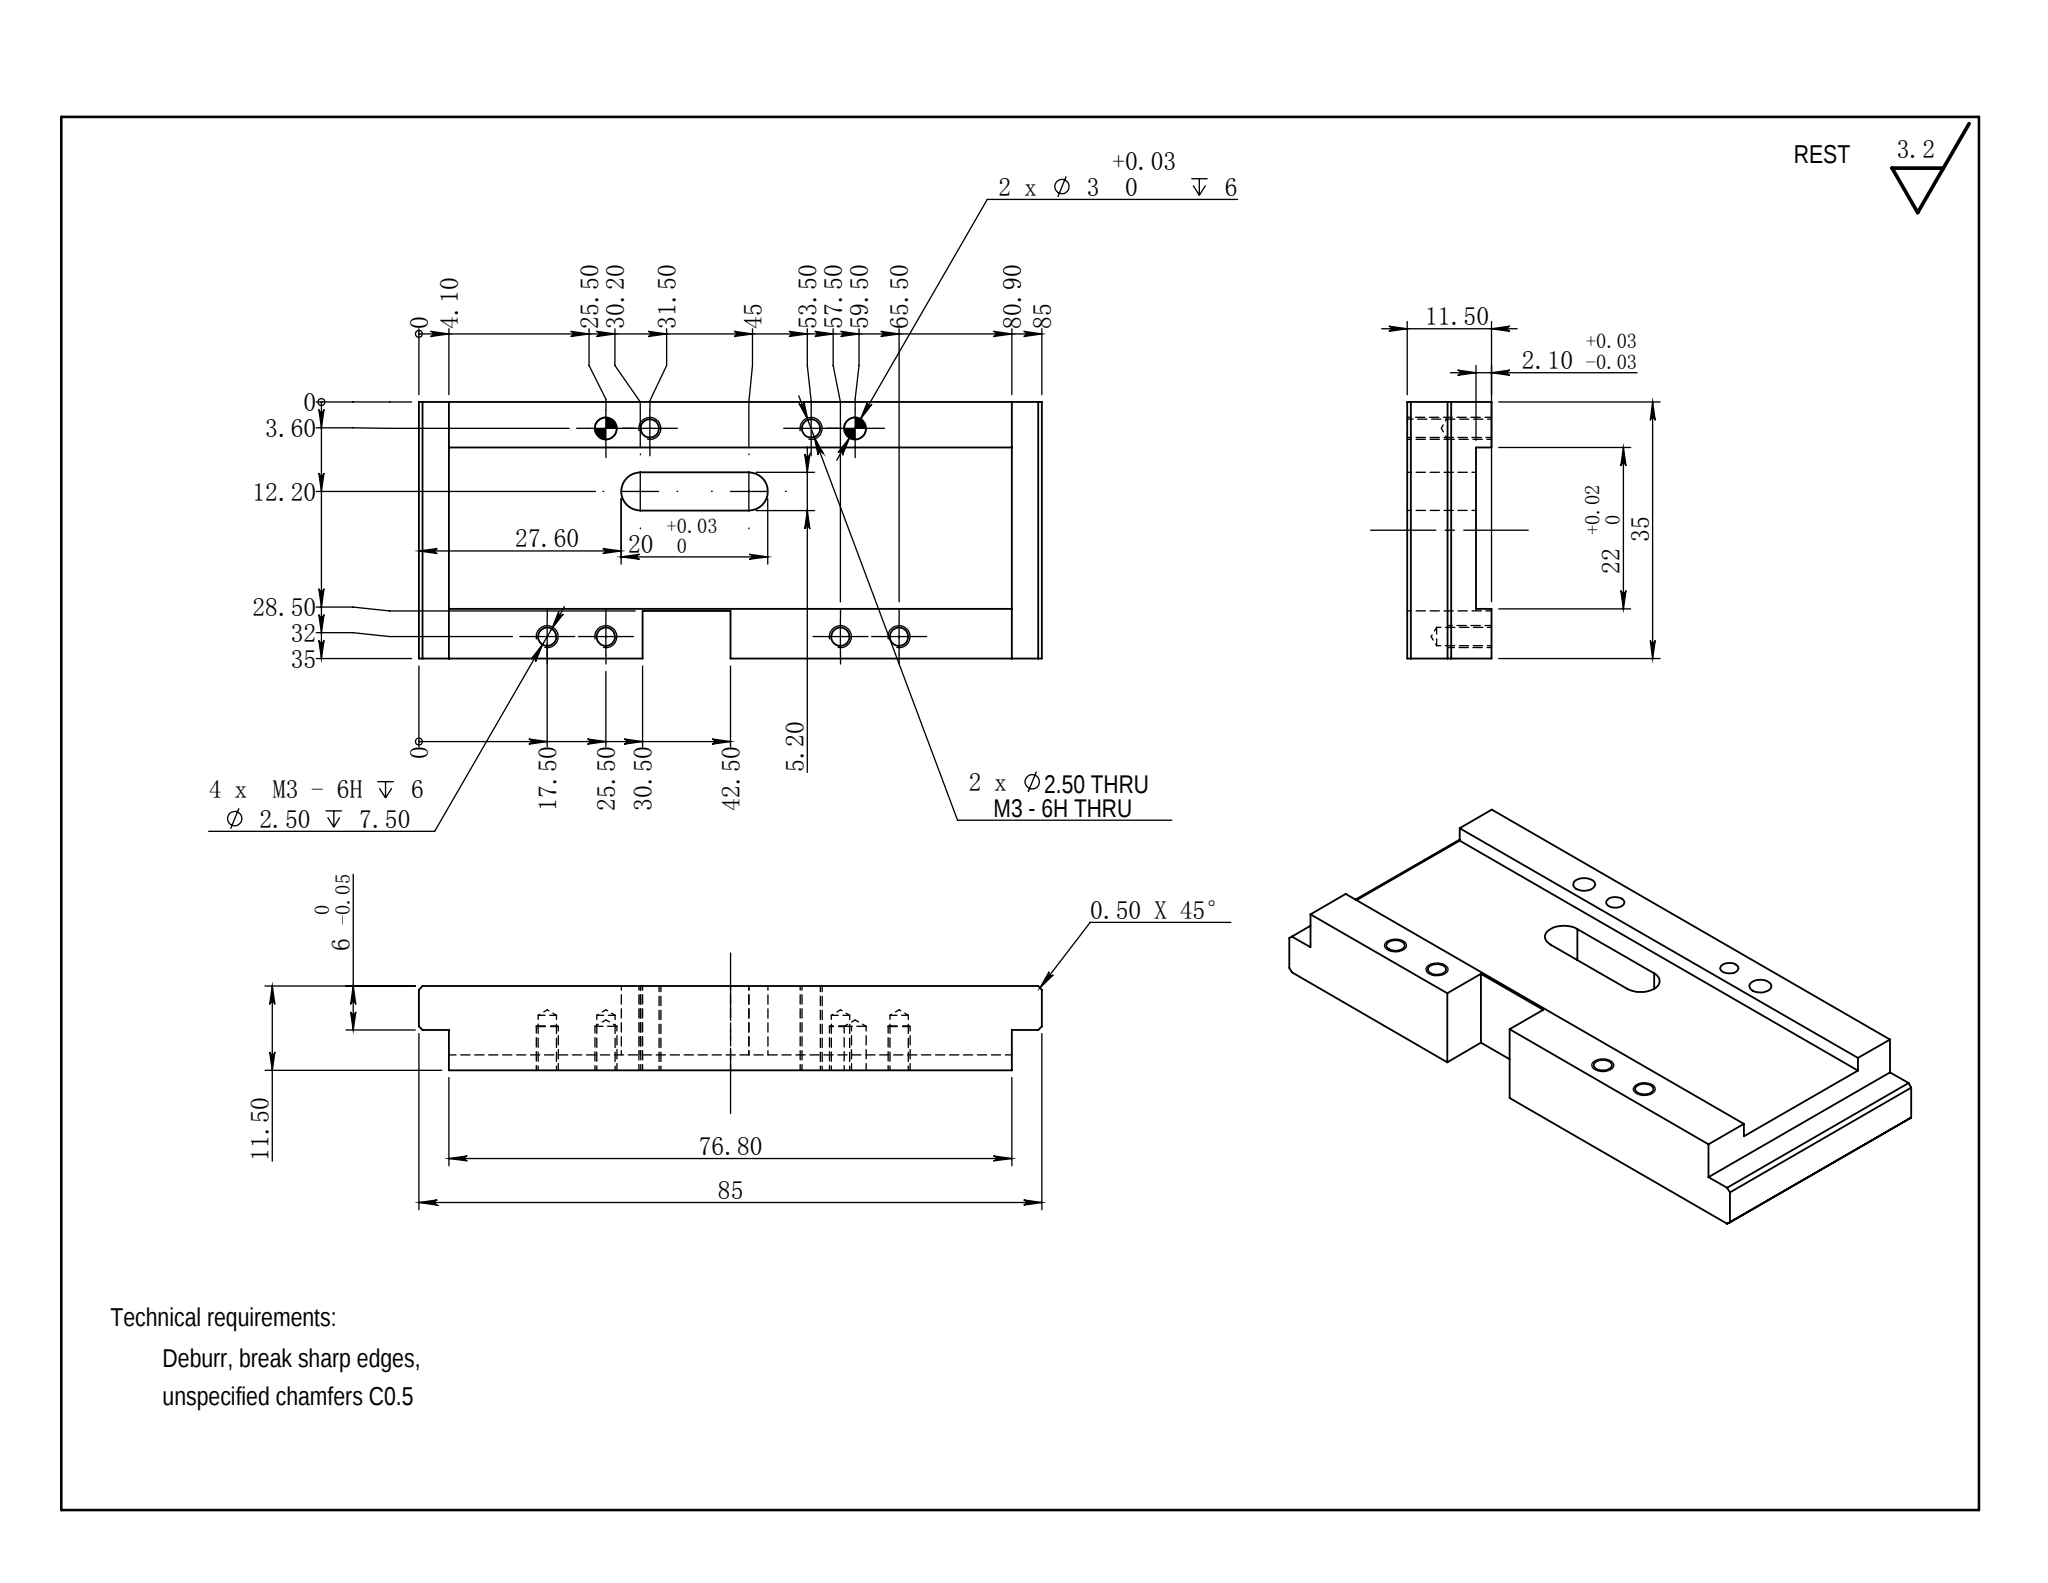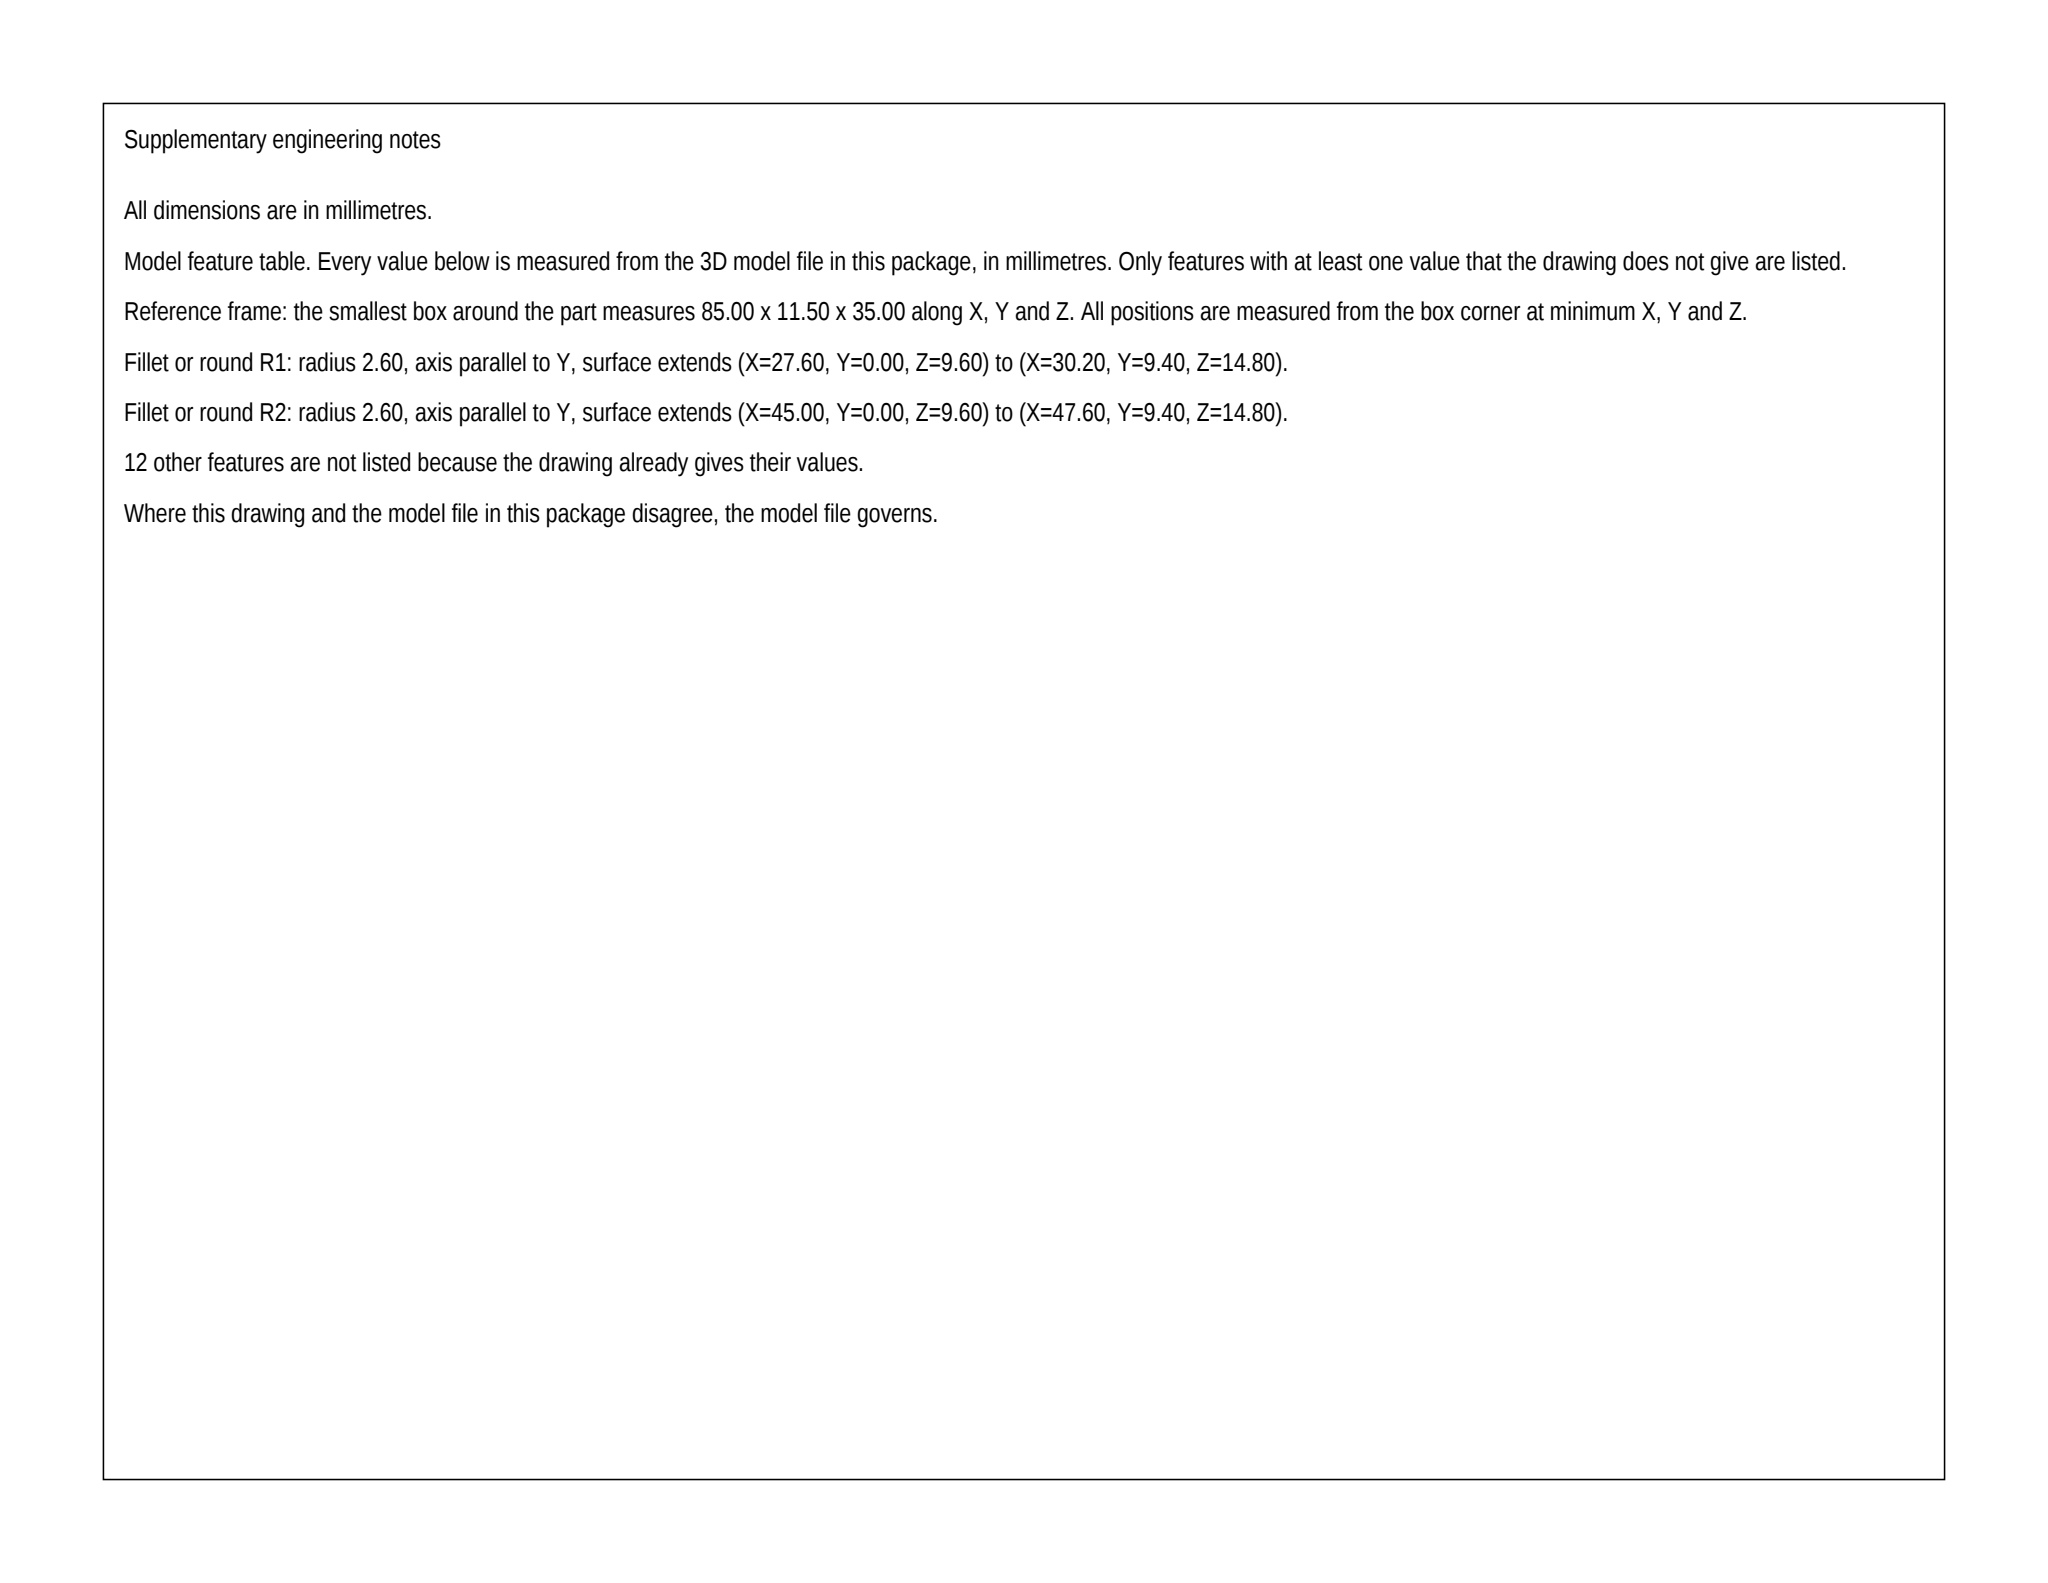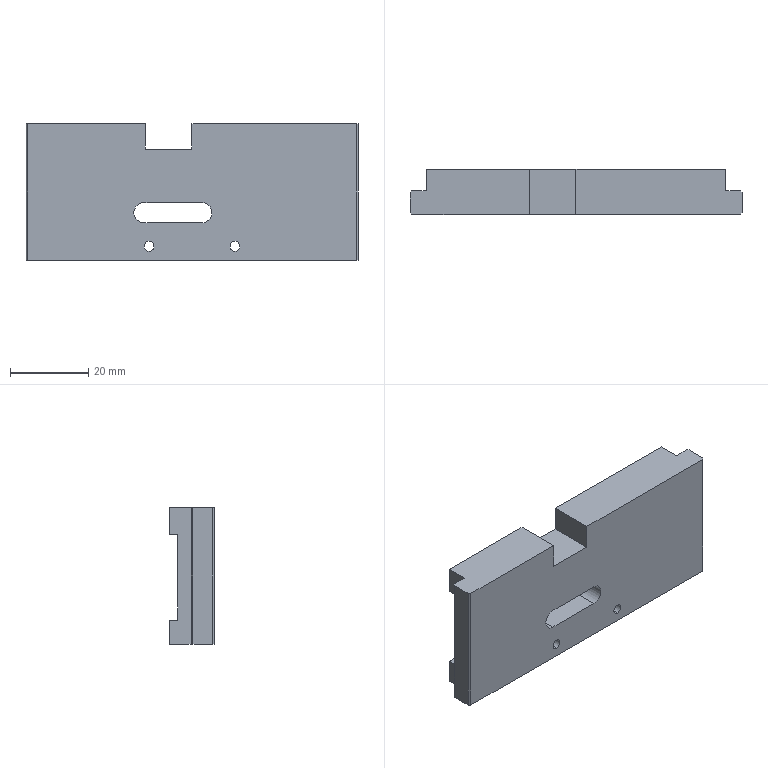Part | SolidWorks | mm | 1 solid | 54 faces | box 85 x 11.5 x 35 mm | volume 26894 mm3 | plane 24 | cylinder 18 | cone 12 | commonest cylinder face diameters 2.5 x12 3 x4 5.2 x2
Drawing notes:
22 GROOVE 6.20 FROM 0 DATUM EDGE, 6.80 FROM 35 EDGE | from the solid: z-planes 6.2 and 28.2 bound 22 wide groove in 35 width; 35-28.2=6.8
CENTRAL SLOT 5.20 WIDE, R2.60 ENDS, DP 9.40 | from the solid: 2x cyl Ø5.2 axis y at x=30.2 & 45.0, z=12.2, len 9.4; centers 14.8 apart = 20 OA
build123d program:
from build123d import *

# Parameters (mm, degrees)
SKETCH1_W                    = 85
SKETCH1_H                    = 35
BOSS_EXTRUDE1_DEPTH          = 11.5
SKETCH2_W                    = 85
SKETCH2_H                    = 22
CUT_EXTRUDE1_DEPTH           = 2.1
SKETCH4_W                    = 12
SKETCH4_H                    = 6.5
CUT_EXTRUDE3_DEPTH           = 48.379
M3_TAPPED_HOLE1_D            = 2.5
M3_TAPPED_HOLE1_DEPTH        = 7.5
M3_TAPPED_HOLE1_TIP          = 0.7511
M3_TAPPED_HOLE2_D            = 2.5
SKETCH27_W                   = 4.1
SKETCH27_H                   = 35
CUT_EXTRUDE9_DEPTH           = 5.5
F_3_0_3_DIAMETER_HOLE1_D     = 3
F_3_0_3_DIAMETER_HOLE1_DEPTH = 6
F_3_0_3_DIAMETER_HOLE1_TIP   = 0.866
SKETCH30_R                   = 2.6
CUT_EXTRUDE10_DEPTH          = 47.913
CHAMFER3_SIZE                = 0.5
CUT_EXTRUDE12_REACH          = 48.913


with BuildPart() as part:
    # Sketch1 → Boss-Extrude1 (new body)
    with BuildSketch(Plane(origin=(0, 0, 0), x_dir=(1, 0, 0), z_dir=(0, 1, 0))):
        Rectangle(SKETCH1_W, SKETCH1_H)
    extrude(amount=BOSS_EXTRUDE1_DEPTH)

    # Sketch2 → Cut-Extrude1 (cut)
    with BuildSketch(Plane(origin=(0, 11.5, 0), x_dir=(1, 0, 0), z_dir=(0, 1, 0))):
        with Locations((0, 0.3)):
            Rectangle(SKETCH2_W, SKETCH2_H)
    extrude(amount=-CUT_EXTRUDE1_DEPTH, mode=Mode.SUBTRACT)

    # Sketch4 → Cut-Extrude3 (cut, through all)
    with BuildSketch(Plane(origin=(0, 11.5, 0), x_dir=(1, 0, 0), z_dir=(0, 1, 0))):
        with Locations((-6, -14.25)):
            Rectangle(SKETCH4_W, SKETCH4_H)
    extrude(amount=-CUT_EXTRUDE3_DEPTH, mode=Mode.SUBTRACT)

    # M3 Tapped Hole1
    with Locations(Plane(origin=(0, 11.5, 0), x_dir=(1, 0, 0), z_dir=(0, 1, 0))):
        with Locations((-25, -14.5), (-17, -14.5), (15, -14.5), (23, -14.5)):
            Hole(M3_TAPPED_HOLE1_D / 2, depth=M3_TAPPED_HOLE1_DEPTH)
            with Locations((0, 0, -(M3_TAPPED_HOLE1_DEPTH + M3_TAPPED_HOLE1_TIP / 2))):  # 118° drill point
                Cone(0, M3_TAPPED_HOLE1_D / 2, M3_TAPPED_HOLE1_TIP, mode=Mode.SUBTRACT)

    # M3 Tapped Hole2 (through all)
    with Locations(Plane(origin=(0, 0, 0), x_dir=(-1, 0, 0), z_dir=(0, -1, 0))):
        with Locations((-11, 13.9), (11, 13.9)):
            Hole(M3_TAPPED_HOLE2_D / 2)

    # Sketch27 → Cut-Extrude9 (cut)
    with BuildSketch(Plane(origin=(0, 11.5, 0), x_dir=(1, 0, 0), z_dir=(0, 1, 0))):
        with Locations((-40.45, 0)):
            Rectangle(SKETCH27_W, SKETCH27_H)
        with Locations((40.45, 0)):
            Rectangle(SKETCH27_W, SKETCH27_H)
    extrude(amount=-CUT_EXTRUDE9_DEPTH, mode=Mode.SUBTRACT)

    # 3.0 _3_ Diameter Hole1
    with Locations(Plane(origin=(0, 11.5, 0), x_dir=(1, 0, 0), z_dir=(0, 1, 0))):
        with Locations((-17, 13.9), (17, 13.9)):
            Hole(F_3_0_3_DIAMETER_HOLE1_D / 2, depth=F_3_0_3_DIAMETER_HOLE1_DEPTH)
            with Locations((0, 0, -(F_3_0_3_DIAMETER_HOLE1_DEPTH + F_3_0_3_DIAMETER_HOLE1_TIP / 2))):  # 120° drill point
                Cone(0, F_3_0_3_DIAMETER_HOLE1_D / 2, F_3_0_3_DIAMETER_HOLE1_TIP, mode=Mode.SUBTRACT)

    # Sketch30 → Cut-Extrude10 (cut, through all)
    with BuildSketch(Plane(origin=(0, 9.4, 0), x_dir=(1, 0, 0), z_dir=(0, 1, 0))):
        with Locations(Location((-12.3, 5.3, 0), (0, 0, 270))):
            Circle(SKETCH30_R)
        with Locations(Location((2.5, 5.3, 0), (0, 0, 270))):
            Circle(SKETCH30_R)
    extrude(amount=-CUT_EXTRUDE10_DEPTH, mode=Mode.SUBTRACT)

    # Chamfer3
    chamfer3_edges = [part.edges().sort_by_distance(p)[0] for p in [
        (42.5, 6, 0),
        (42.5, 0, 0),
        (-42.5, 0, 0),
        (-42.5, 6, 0),
    ]]
    chamfer(chamfer3_edges, length=CHAMFER3_SIZE)

    # Sketch32 → Cut-Extrude12 (cut, up to next)
    with BuildSketch(Plane(origin=(0, 9.4, 0), x_dir=(1, 0, 0), z_dir=(0, 1, 0)), mode=Mode.PRIVATE) as cut_extrude12_sk1:
        with BuildLine():
            Line((-12.3, 7.9), (2.5, 7.9))
            ThreePointArc((2.5, 7.9), (5.1, 5.3), (2.5, 2.7))
            Line((2.5, 2.7), (-12.3, 2.7))
            ThreePointArc((-12.3, 2.7), (-14.9, 5.3), (-12.3, 7.9))
        make_face()
    cut_extrude12_tool1 = extrude(cut_extrude12_sk1.sketch, amount=-CUT_EXTRUDE12_REACH, mode=Mode.PRIVATE) & part.part
    add(cut_extrude12_tool1.solids().sort_by_distance((-4.9, 9.4, -5.3))[0], mode=Mode.SUBTRACT)


solid = part.part